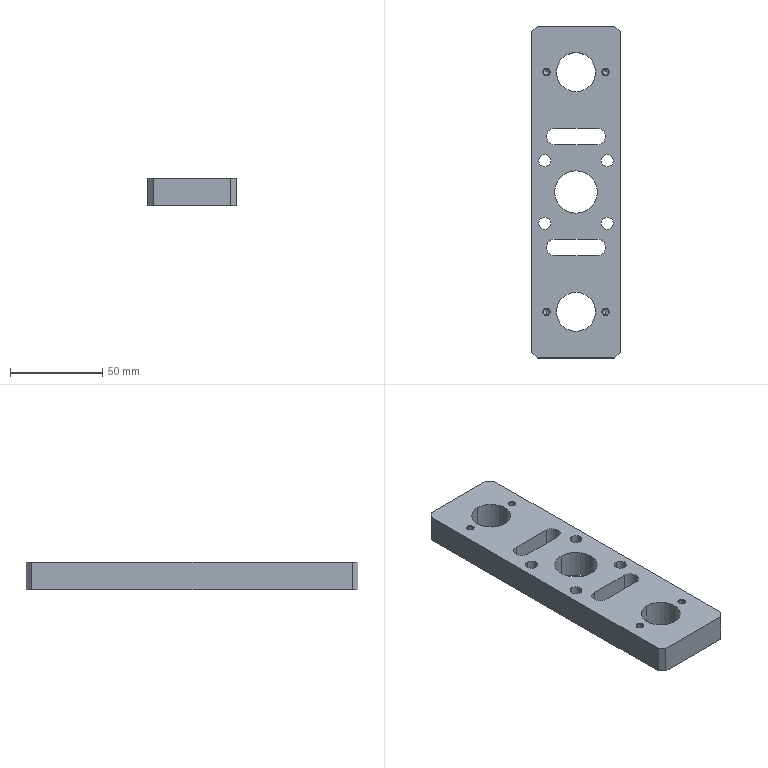Component | SolidWorks | DirectPressureVerticalSeal-1_CylinderFixingPlate-1 | 1 solid | 68 faces | box 48 x 180 x 15 mm | volume 99943 mm3 | cylinder 34 | plane 18 | cone 16 | commonest cylinder face diameters 11 x8 6.5 x8 3.3 x8 21.2 x4 9 x4 23 x2
build123d program:
from build123d import *

# Parameters (mm, degrees)
SKETCH1_W                                            = 180
SKETCH1_H                                            = 48
BOSS_EXTRUDE1_DEPTH                                  = 15
CUT_EXTRUDE1_DEPTH                                   = 95.345
CUT_EXTRUDE2_DEPTH                                   = 95.345
F_23_0_23_DIAMETER_HOLE1_D                           = 23
M20_CLEARANCE_HOLE1_D                                = 21.2
F_3_3_3_3_DIAMETER_HOLE1_D                           = 3.3
F_3_3_3_3_DIAMETER_HOLE1_DEPTH                       = 13.5
F_3_3_3_3_DIAMETER_HOLE1_TIP                         = 0.9914
CYLINDRICAL_COUNTERSUNK_HOLE_1_FOR_M6_HE_D           = 6.5
CYLINDRICAL_COUNTERSUNK_HOLE_1_FOR_M6_HE_CBORE_D     = 11
CYLINDRICAL_COUNTERSUNK_HOLE_1_FOR_M6_HE_CBORE_DEPTH = 8
CHAMFER1_SIZE                                        = 3
CHAMFER2_SIZE                                        = 0.375


with BuildPart() as part:
    # Sketch1 → Boss-Extrude1 (new body)
    with BuildSketch(Plane(origin=(0, 0, -7.5), x_dir=(-1, 0, 0), z_dir=(0, 0, -1))):
        Rectangle(SKETCH1_W, SKETCH1_H)
    extrude(amount=-BOSS_EXTRUDE1_DEPTH)

    # Sketch2 → Cut-Extrude1 (cut, through all)
    with BuildSketch(Plane(origin=(0, 0, -7.5), x_dir=(-1, 0, 0), z_dir=(0, 0, -1))):
        with BuildLine():
            Line((-25.5, -11.5), (-25.5, 11.5))
            ThreePointArc((-25.5, 11.5), (-30, 16), (-34.5, 11.5))
            Line((-34.5, 11.5), (-34.5, -11.5))
            ThreePointArc((-34.5, -11.5), (-30, -16), (-25.5, -11.5))
        make_face()
    extrude(amount=-CUT_EXTRUDE1_DEPTH, mode=Mode.SUBTRACT)

    # Sketch3 → Cut-Extrude2 (cut, through all)
    with BuildSketch(Plane.XY.offset(7.5)):
        with BuildLine():
            Line((-25.5, -11.5), (-25.5, 11.5))
            ThreePointArc((-25.5, 11.5), (-30, 16), (-34.5, 11.5))
            Line((-34.5, 11.5), (-34.5, -11.5))
            ThreePointArc((-34.5, -11.5), (-30, -16), (-25.5, -11.5))
        make_face()
    extrude(amount=-CUT_EXTRUDE2_DEPTH, mode=Mode.SUBTRACT)

    # 23.0 _23_ Diameter Hole1 (through all)
    with Locations(Plane.XY.offset(7.5)):
        with Locations((0, 0)):
            Hole(F_23_0_23_DIAMETER_HOLE1_D / 2)

    # M20 Clearance Hole1 (through all)
    with Locations(Plane.XY.offset(7.5)):
        with Locations((65, 0), (-65, 0)):
            Hole(M20_CLEARANCE_HOLE1_D / 2)

    # 3.3 _3.3_ Diameter Hole1
    with Locations(Plane.XY.offset(7.5)):
        with Locations((65, -16), (65, 16), (-65, -16), (-65, 16)):
            Hole(F_3_3_3_3_DIAMETER_HOLE1_D / 2, depth=F_3_3_3_3_DIAMETER_HOLE1_DEPTH)
            with Locations((0, 0, -(F_3_3_3_3_DIAMETER_HOLE1_DEPTH + F_3_3_3_3_DIAMETER_HOLE1_TIP / 2))):  # 118° drill point
                Cone(0, F_3_3_3_3_DIAMETER_HOLE1_D / 2, F_3_3_3_3_DIAMETER_HOLE1_TIP, mode=Mode.SUBTRACT)

    # Cylindrical Countersunk Hole 1 for M6 He (through all)
    with Locations(Plane(origin=(0, 0, -7.5), x_dir=(-1, 0, 0), z_dir=(0, 0, -1))):
        with Locations((17, 17), (17, -17), (-17, -17), (-17, 17)):
            CounterBoreHole(CYLINDRICAL_COUNTERSUNK_HOLE_1_FOR_M6_HE_D / 2, CYLINDRICAL_COUNTERSUNK_HOLE_1_FOR_M6_HE_CBORE_D / 2, CYLINDRICAL_COUNTERSUNK_HOLE_1_FOR_M6_HE_CBORE_DEPTH)

    # Chamfer1
    chamfer1_edges = [part.edges().sort_by_distance(p)[0] for p in [
        (-90, 24, 0),
        (-90, -24, 0),
        (90, -24, 0),
        (90, 24, 0),
    ]]
    chamfer(chamfer1_edges, length=CHAMFER1_SIZE)

    # Chamfer2
    chamfer2_edges = [part.edges().sort_by_distance(p)[0] for p in [
        (-63.35, 16, 7.5),
        (-63.35, -16, 7.5),
        (66.65, 16, 7.5),
        (66.65, -16, 7.5),
    ]]
    chamfer(chamfer2_edges, length=CHAMFER2_SIZE)


solid = part.part

# Placed as in the assembly
solid = solid.moved(Location((-298.746, 246.873, 311), (0, 0, 90)))